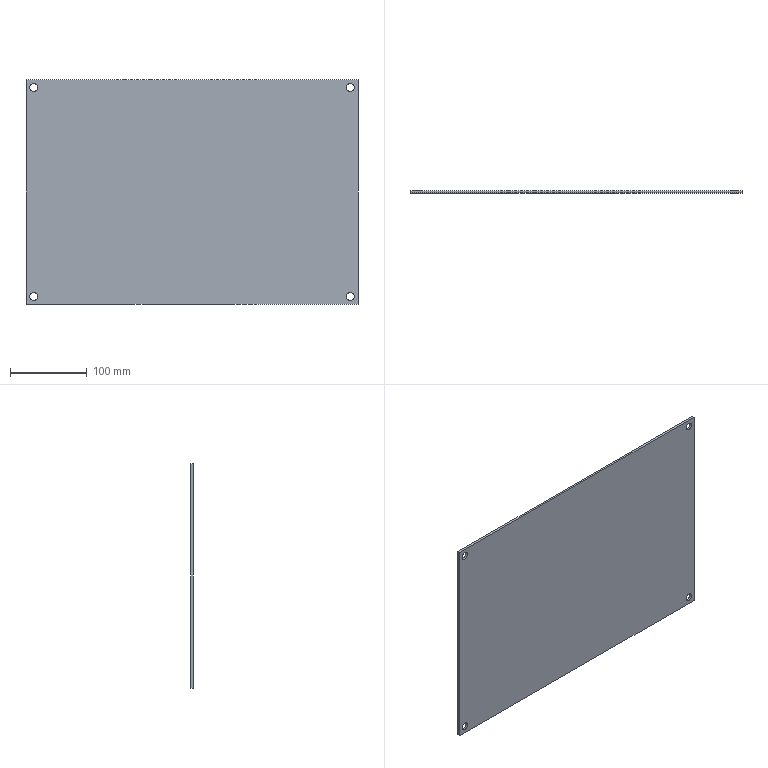Component | SolidWorks | FuelTank-1_FuelTankCap-1 | 1 solid | 14 faces | box 432 x 3 x 292 mm | volume 377490 mm3 | cylinder 8 | plane 6 | commonest cylinder face diameters 10 x8
build123d program:
from build123d import *

# Parameters (mm, degrees)
SKETCH1_W           = 432
SKETCH1_H           = 292
BOSS_EXTRUDE1_DEPTH = 3
SKETCH2_R           = 5
CUT_EXTRUDE1_DEPTH  = 3


with BuildPart() as part:
    # Sketch1 → Boss-Extrude1 (new body)
    with BuildSketch(Plane.XY):
        with Locations((151.422, -114.636)):
            Rectangle(SKETCH1_W, SKETCH1_H)
    extrude(amount=BOSS_EXTRUDE1_DEPTH)

    # Sketch2 → Cut-Extrude1 (cut)
    with BuildSketch(Plane.XY.offset(3)):
        with Locations((-54.578, 21.364)):
            Circle(SKETCH2_R)
        with Locations((357.422, 21.364)):
            Circle(SKETCH2_R)
        with Locations((357.422, -250.636)):
            Circle(SKETCH2_R)
        with Locations((-54.578, -250.636)):
            Circle(SKETCH2_R)
    extrude(amount=-CUT_EXTRUDE1_DEPTH, mode=Mode.SUBTRACT)


solid = part.part

# Placed as in the assembly
solid = solid.moved(Location((34.029, -468.434, -406.883), (90, 0, 0)))
STEP:
#1=CARTESIAN_POINT('',(-1.006,-18.442,-25.887));
#2=VERTEX_POINT('',#1);
#3=CARTESIAN_POINT('',(-0.6122,-18.442,-25.887));
#4=VERTEX_POINT('',#3);
#5=CARTESIAN_POINT('',(-0.809,-18.442,-25.887));
#6=DIRECTION('',(0.,-1.,-0.));
#7=DIRECTION('',(1.,0.,0.));
#8=AXIS2_PLACEMENT_3D('',#5,#6,#7);
#9=CIRCLE('',#8,0.1969);
#10=EDGE_CURVE('',#2,#4,#9,.T.);
#11=ORIENTED_EDGE('',*,*,#10,.F.);
#12=CARTESIAN_POINT('',(-1.006,-18.56,-25.887));
#13=VERTEX_POINT('',#12);
#14=CARTESIAN_POINT('',(-1.006,-18.442,-25.887));
#15=DIRECTION('',(0.,-1.,-0.));
#16=VECTOR('',#15,39.37);
#17=LINE('',#14,#16);
#18=EDGE_CURVE('',#2,#13,#17,.T.);
#19=ORIENTED_EDGE('',*,*,#18,.T.);
#20=CARTESIAN_POINT('',(-0.6122,-18.56,-25.887));
#21=VERTEX_POINT('',#20);
#22=CARTESIAN_POINT('',(-0.809,-18.56,-25.887));
#23=DIRECTION('',(0.,-1.,-0.));
#24=DIRECTION('',(1.,0.,0.));
#25=AXIS2_PLACEMENT_3D('',#22,#23,#24);
#26=CIRCLE('',#25,0.1969);
#27=EDGE_CURVE('',#13,#21,#26,.T.);
#28=ORIENTED_EDGE('',*,*,#27,.T.);
#29=CARTESIAN_POINT('',(-0.6122,-18.442,-25.887));
#30=DIRECTION('',(0.,-1.,-0.));
#31=VECTOR('',#30,39.37);
#32=LINE('',#29,#31);
#33=EDGE_CURVE('',#4,#21,#32,.T.);
#34=ORIENTED_EDGE('',*,*,#33,.F.);
#35=EDGE_LOOP('',(#11,#19,#28,#34));
#36=FACE_OUTER_BOUND('',#35,.T.);
#37=CARTESIAN_POINT('',(-0.809,-18.442,-25.887));
#38=DIRECTION('',(0.,-1.,-0.));
#39=DIRECTION('',(1.,0.,0.));
#40=AXIS2_PLACEMENT_3D('',#37,#38,#39);
#41=CYLINDRICAL_SURFACE('',#40,0.1969);
#42=ADVANCED_FACE('',(#36),#41,.F.);
#43=CARTESIAN_POINT('',(15.215,-18.442,-25.887));
#44=VERTEX_POINT('',#43);
#45=CARTESIAN_POINT('',(15.608,-18.442,-25.887));
#46=VERTEX_POINT('',#45);
#47=CARTESIAN_POINT('',(15.411,-18.442,-25.887));
#48=DIRECTION('',(0.,-1.,-0.));
#49=DIRECTION('',(1.,0.,0.));
#50=AXIS2_PLACEMENT_3D('',#47,#48,#49);
#51=CIRCLE('',#50,0.1969);
#52=EDGE_CURVE('',#44,#46,#51,.T.);
#53=ORIENTED_EDGE('',*,*,#52,.F.);
#54=CARTESIAN_POINT('',(15.215,-18.56,-25.887));
#55=VERTEX_POINT('',#54);
#56=CARTESIAN_POINT('',(15.215,-18.442,-25.887));
#57=DIRECTION('',(0.,-1.,-0.));
#58=VECTOR('',#57,39.37);
#59=LINE('',#56,#58);
#60=EDGE_CURVE('',#44,#55,#59,.T.);
#61=ORIENTED_EDGE('',*,*,#60,.T.);
#62=CARTESIAN_POINT('',(15.608,-18.56,-25.887));
#63=VERTEX_POINT('',#62);
#64=CARTESIAN_POINT('',(15.411,-18.56,-25.887));
#65=DIRECTION('',(0.,-1.,-0.));
#66=DIRECTION('',(1.,0.,0.));
#67=AXIS2_PLACEMENT_3D('',#64,#65,#66);
#68=CIRCLE('',#67,0.1969);
#69=EDGE_CURVE('',#55,#63,#68,.T.);
#70=ORIENTED_EDGE('',*,*,#69,.T.);
#71=CARTESIAN_POINT('',(15.608,-18.442,-25.887));
#72=DIRECTION('',(0.,-1.,-0.));
#73=VECTOR('',#72,39.37);
#74=LINE('',#71,#73);
#75=EDGE_CURVE('',#46,#63,#74,.T.);
#76=ORIENTED_EDGE('',*,*,#75,.F.);
#77=EDGE_LOOP('',(#53,#61,#70,#76));
#78=FACE_OUTER_BOUND('',#77,.T.);
#79=CARTESIAN_POINT('',(15.411,-18.442,-25.887));
#80=DIRECTION('',(0.,-1.,-0.));
#81=DIRECTION('',(1.,0.,0.));
#82=AXIS2_PLACEMENT_3D('',#79,#80,#81);
#83=CYLINDRICAL_SURFACE('',#82,0.1969);
#84=ADVANCED_FACE('',(#78),#83,.F.);
#85=CARTESIAN_POINT('',(15.215,-18.442,-15.178));
#86=VERTEX_POINT('',#85);
#87=CARTESIAN_POINT('',(15.608,-18.442,-15.178));
#88=VERTEX_POINT('',#87);
#89=CARTESIAN_POINT('',(15.411,-18.442,-15.178));
#90=DIRECTION('',(0.,-1.,-0.));
#91=DIRECTION('',(1.,0.,0.));
#92=AXIS2_PLACEMENT_3D('',#89,#90,#91);
#93=CIRCLE('',#92,0.1969);
#94=EDGE_CURVE('',#86,#88,#93,.T.);
#95=ORIENTED_EDGE('',*,*,#94,.F.);
#96=CARTESIAN_POINT('',(15.215,-18.56,-15.178));
#97=VERTEX_POINT('',#96);
#98=CARTESIAN_POINT('',(15.215,-18.442,-15.178));
#99=DIRECTION('',(0.,-1.,-0.));
#100=VECTOR('',#99,39.37);
#101=LINE('',#98,#100);
#102=EDGE_CURVE('',#86,#97,#101,.T.);
#103=ORIENTED_EDGE('',*,*,#102,.T.);
#104=CARTESIAN_POINT('',(15.608,-18.56,-15.178));
#105=VERTEX_POINT('',#104);
#106=CARTESIAN_POINT('',(15.411,-18.56,-15.178));
#107=DIRECTION('',(0.,-1.,-0.));
#108=DIRECTION('',(1.,0.,0.));
#109=AXIS2_PLACEMENT_3D('',#106,#107,#108);
#110=CIRCLE('',#109,0.1969);
#111=EDGE_CURVE('',#97,#105,#110,.T.);
#112=ORIENTED_EDGE('',*,*,#111,.T.);
#113=CARTESIAN_POINT('',(15.608,-18.442,-15.178));
#114=DIRECTION('',(0.,-1.,-0.));
#115=VECTOR('',#114,39.37);
#116=LINE('',#113,#115);
#117=EDGE_CURVE('',#88,#105,#116,.T.);
#118=ORIENTED_EDGE('',*,*,#117,.F.);
#119=EDGE_LOOP('',(#95,#103,#112,#118));
#120=FACE_OUTER_BOUND('',#119,.T.);
#121=CARTESIAN_POINT('',(15.411,-18.442,-15.178));
#122=DIRECTION('',(0.,-1.,-0.));
#123=DIRECTION('',(1.,0.,0.));
#124=AXIS2_PLACEMENT_3D('',#121,#122,#123);
#125=CYLINDRICAL_SURFACE('',#124,0.1969);
#126=ADVANCED_FACE('',(#120),#125,.F.);
#127=CARTESIAN_POINT('',(-1.006,-18.442,-15.178));
#128=VERTEX_POINT('',#127);
#129=CARTESIAN_POINT('',(-0.6122,-18.442,-15.178));
#130=VERTEX_POINT('',#129);
#131=CARTESIAN_POINT('',(-0.809,-18.442,-15.178));
#132=DIRECTION('',(0.,-1.,-0.));
#133=DIRECTION('',(1.,0.,0.));
#134=AXIS2_PLACEMENT_3D('',#131,#132,#133);
#135=CIRCLE('',#134,0.1969);
#136=EDGE_CURVE('',#128,#130,#135,.T.);
#137=ORIENTED_EDGE('',*,*,#136,.F.);
#138=CARTESIAN_POINT('',(-1.006,-18.56,-15.178));
#139=VERTEX_POINT('',#138);
#140=CARTESIAN_POINT('',(-1.006,-18.442,-15.178));
#141=DIRECTION('',(0.,-1.,-0.));
#142=VECTOR('',#141,39.37);
#143=LINE('',#140,#142);
#144=EDGE_CURVE('',#128,#139,#143,.T.);
#145=ORIENTED_EDGE('',*,*,#144,.T.);
#146=CARTESIAN_POINT('',(-0.6122,-18.56,-15.178));
#147=VERTEX_POINT('',#146);
#148=CARTESIAN_POINT('',(-0.809,-18.56,-15.178));
#149=DIRECTION('',(0.,-1.,-0.));
#150=DIRECTION('',(1.,0.,0.));
#151=AXIS2_PLACEMENT_3D('',#148,#149,#150);
#152=CIRCLE('',#151,0.1969);
#153=EDGE_CURVE('',#139,#147,#152,.T.);
#154=ORIENTED_EDGE('',*,*,#153,.T.);
#155=CARTESIAN_POINT('',(-0.6122,-18.442,-15.178));
#156=DIRECTION('',(0.,-1.,-0.));
#157=VECTOR('',#156,39.37);
#158=LINE('',#155,#157);
#159=EDGE_CURVE('',#130,#147,#158,.T.);
#160=ORIENTED_EDGE('',*,*,#159,.F.);
#161=EDGE_LOOP('',(#137,#145,#154,#160));
#162=FACE_OUTER_BOUND('',#161,.T.);
#163=CARTESIAN_POINT('',(-0.809,-18.442,-15.178));
#164=DIRECTION('',(0.,-1.,-0.));
#165=DIRECTION('',(1.,0.,0.));
#166=AXIS2_PLACEMENT_3D('',#163,#164,#165);
#167=CYLINDRICAL_SURFACE('',#166,0.1969);
#168=ADVANCED_FACE('',(#162),#167,.F.);
#169=CARTESIAN_POINT('',(-1.203,-18.442,-14.784));
#170=VERTEX_POINT('',#169);
#171=CARTESIAN_POINT('',(-1.203,-18.442,-26.28));
#172=VERTEX_POINT('',#171);
#173=CARTESIAN_POINT('',(-1.203,-18.442,-14.784));
#174=DIRECTION('',(0.,0.,-1.));
#175=VECTOR('',#174,39.37);
#176=LINE('',#173,#175);
#177=EDGE_CURVE('',#170,#172,#176,.T.);
#178=ORIENTED_EDGE('',*,*,#177,.T.);
#179=CARTESIAN_POINT('',(-1.203,-18.56,-26.28));
#180=VERTEX_POINT('',#179);
#181=CARTESIAN_POINT('',(-1.203,-18.56,-26.28));
#182=DIRECTION('',(-0.,1.,0.));
#183=VECTOR('',#182,39.37);
#184=LINE('',#181,#183);
#185=EDGE_CURVE('',#180,#172,#184,.T.);
#186=ORIENTED_EDGE('',*,*,#185,.F.);
#187=CARTESIAN_POINT('',(-1.203,-18.56,-14.784));
#188=VERTEX_POINT('',#187);
#189=CARTESIAN_POINT('',(-1.203,-18.56,-14.784));
#190=DIRECTION('',(0.,0.,-1.));
#191=VECTOR('',#190,39.37);
#192=LINE('',#189,#191);
#193=EDGE_CURVE('',#188,#180,#192,.T.);
#194=ORIENTED_EDGE('',*,*,#193,.F.);
#195=CARTESIAN_POINT('',(-1.203,-18.56,-14.784));
#196=DIRECTION('',(-0.,1.,0.));
#197=VECTOR('',#196,39.37);
#198=LINE('',#195,#197);
#199=EDGE_CURVE('',#188,#170,#198,.T.);
#200=ORIENTED_EDGE('',*,*,#199,.T.);
#201=EDGE_LOOP('',(#178,#186,#194,#200));
#202=FACE_OUTER_BOUND('',#201,.T.);
#203=CARTESIAN_POINT('',(-1.203,-18.56,-14.784));
#204=DIRECTION('',(1.,0.,0.));
#205=DIRECTION('',(-0.,-0.,1.));
#206=AXIS2_PLACEMENT_3D('',#203,#204,#205);
#207=PLANE('',#206);
#208=ADVANCED_FACE('',(#202),#207,.F.);
#209=CARTESIAN_POINT('',(15.805,-18.442,-26.28));
#210=VERTEX_POINT('',#209);
#211=CARTESIAN_POINT('',(-1.203,-18.442,-26.28));
#212=DIRECTION('',(1.,0.,0.));
#213=VECTOR('',#212,39.37);
#214=LINE('',#211,#213);
#215=EDGE_CURVE('',#172,#210,#214,.T.);
#216=ORIENTED_EDGE('',*,*,#215,.T.);
#217=CARTESIAN_POINT('',(15.805,-18.56,-26.28));
#218=VERTEX_POINT('',#217);
#219=CARTESIAN_POINT('',(15.805,-18.56,-26.28));
#220=DIRECTION('',(-0.,1.,0.));
#221=VECTOR('',#220,39.37);
#222=LINE('',#219,#221);
#223=EDGE_CURVE('',#218,#210,#222,.T.);
#224=ORIENTED_EDGE('',*,*,#223,.F.);
#225=CARTESIAN_POINT('',(-1.203,-18.56,-26.28));
#226=DIRECTION('',(1.,0.,0.));
#227=VECTOR('',#226,39.37);
#228=LINE('',#225,#227);
#229=EDGE_CURVE('',#180,#218,#228,.T.);
#230=ORIENTED_EDGE('',*,*,#229,.F.);
#231=ORIENTED_EDGE('',*,*,#185,.T.);
#232=EDGE_LOOP('',(#216,#224,#230,#231));
#233=FACE_OUTER_BOUND('',#232,.T.);
#234=CARTESIAN_POINT('',(-1.203,-18.56,-26.28));
#235=DIRECTION('',(-0.,-0.,1.));
#236=DIRECTION('',(0.,-1.,-0.));
#237=AXIS2_PLACEMENT_3D('',#234,#235,#236);
#238=PLANE('',#237);
#239=ADVANCED_FACE('',(#233),#238,.F.);
#240=CARTESIAN_POINT('',(15.805,-18.442,-14.784));
#241=VERTEX_POINT('',#240);
#242=CARTESIAN_POINT('',(15.805,-18.442,-14.784));
#243=DIRECTION('',(-0.,-0.,1.));
#244=VECTOR('',#243,39.37);
#245=LINE('',#242,#244);
#246=EDGE_CURVE('',#210,#241,#245,.T.);
#247=ORIENTED_EDGE('',*,*,#246,.T.);
#248=CARTESIAN_POINT('',(15.805,-18.56,-14.784));
#249=VERTEX_POINT('',#248);
#250=CARTESIAN_POINT('',(15.805,-18.56,-14.784));
#251=DIRECTION('',(-0.,1.,0.));
#252=VECTOR('',#251,39.37);
#253=LINE('',#250,#252);
#254=EDGE_CURVE('',#249,#241,#253,.T.);
#255=ORIENTED_EDGE('',*,*,#254,.F.);
#256=CARTESIAN_POINT('',(15.805,-18.56,-14.784));
#257=DIRECTION('',(-0.,-0.,1.));
#258=VECTOR('',#257,39.37);
#259=LINE('',#256,#258);
#260=EDGE_CURVE('',#218,#249,#259,.T.);
#261=ORIENTED_EDGE('',*,*,#260,.F.);
#262=ORIENTED_EDGE('',*,*,#223,.T.);
#263=EDGE_LOOP('',(#247,#255,#261,#262));
#264=FACE_OUTER_BOUND('',#263,.T.);
#265=CARTESIAN_POINT('',(15.805,-18.56,-14.784));
#266=DIRECTION('',(-1.,-0.,-0.));
#267=DIRECTION('',(0.,0.,-1.));
#268=AXIS2_PLACEMENT_3D('',#265,#266,#267);
#269=PLANE('',#268);
#270=ADVANCED_FACE('',(#264),#269,.F.);
#271=CARTESIAN_POINT('',(-1.203,-18.442,-14.784));
#272=DIRECTION('',(-1.,-0.,-0.));
#273=VECTOR('',#272,39.37);
#274=LINE('',#271,#273);
#275=EDGE_CURVE('',#241,#170,#274,.T.);
#276=ORIENTED_EDGE('',*,*,#275,.T.);
#277=ORIENTED_EDGE('',*,*,#199,.F.);
#278=CARTESIAN_POINT('',(-1.203,-18.56,-14.784));
#279=DIRECTION('',(-1.,-0.,-0.));
#280=VECTOR('',#279,39.37);
#281=LINE('',#278,#280);
#282=EDGE_CURVE('',#249,#188,#281,.T.);
#283=ORIENTED_EDGE('',*,*,#282,.F.);
#284=ORIENTED_EDGE('',*,*,#254,.T.);
#285=EDGE_LOOP('',(#276,#277,#283,#284));
#286=FACE_OUTER_BOUND('',#285,.T.);
#287=CARTESIAN_POINT('',(-1.203,-18.56,-14.784));
#288=DIRECTION('',(0.,0.,-1.));
#289=DIRECTION('',(-0.,1.,0.));
#290=AXIS2_PLACEMENT_3D('',#287,#288,#289);
#291=PLANE('',#290);
#292=ADVANCED_FACE('',(#286),#291,.F.);
#293=CARTESIAN_POINT('',(-0.809,-18.56,-25.887));
#294=DIRECTION('',(0.,-1.,-0.));
#295=DIRECTION('',(1.,0.,0.));
#296=AXIS2_PLACEMENT_3D('',#293,#294,#295);
#297=CIRCLE('',#296,0.1969);
#298=EDGE_CURVE('',#21,#13,#297,.T.);
#299=ORIENTED_EDGE('',*,*,#298,.F.);
#300=ORIENTED_EDGE('',*,*,#27,.F.);
#301=EDGE_LOOP('',(#299,#300));
#302=FACE_BOUND('',#301,.T.);
#303=CARTESIAN_POINT('',(15.411,-18.56,-25.887));
#304=DIRECTION('',(0.,-1.,-0.));
#305=DIRECTION('',(1.,0.,0.));
#306=AXIS2_PLACEMENT_3D('',#303,#304,#305);
#307=CIRCLE('',#306,0.1969);
#308=EDGE_CURVE('',#63,#55,#307,.T.);
#309=ORIENTED_EDGE('',*,*,#308,.F.);
#310=ORIENTED_EDGE('',*,*,#69,.F.);
#311=EDGE_LOOP('',(#309,#310));
#312=FACE_BOUND('',#311,.T.);
#313=CARTESIAN_POINT('',(15.411,-18.56,-15.178));
#314=DIRECTION('',(0.,-1.,-0.));
#315=DIRECTION('',(1.,0.,0.));
#316=AXIS2_PLACEMENT_3D('',#313,#314,#315);
#317=CIRCLE('',#316,0.1969);
#318=EDGE_CURVE('',#105,#97,#317,.T.);
#319=ORIENTED_EDGE('',*,*,#318,.F.);
#320=ORIENTED_EDGE('',*,*,#111,.F.);
#321=EDGE_LOOP('',(#319,#320));
#322=FACE_BOUND('',#321,.T.);
#323=CARTESIAN_POINT('',(-0.809,-18.56,-15.178));
#324=DIRECTION('',(0.,-1.,-0.));
#325=DIRECTION('',(1.,0.,0.));
#326=AXIS2_PLACEMENT_3D('',#323,#324,#325);
#327=CIRCLE('',#326,0.1969);
#328=EDGE_CURVE('',#147,#139,#327,.T.);
#329=ORIENTED_EDGE('',*,*,#328,.F.);
#330=ORIENTED_EDGE('',*,*,#153,.F.);
#331=EDGE_LOOP('',(#329,#330));
#332=FACE_BOUND('',#331,.T.);
#333=ORIENTED_EDGE('',*,*,#193,.T.);
#334=ORIENTED_EDGE('',*,*,#229,.T.);
#335=ORIENTED_EDGE('',*,*,#260,.T.);
#336=ORIENTED_EDGE('',*,*,#282,.T.);
#337=EDGE_LOOP('',(#333,#334,#335,#336));
#338=FACE_OUTER_BOUND('',#337,.T.);
#339=CARTESIAN_POINT('',(1.34,-18.56,-16.019));
#340=DIRECTION('',(0.,-1.,-0.));
#341=DIRECTION('',(1.,0.,0.));
#342=AXIS2_PLACEMENT_3D('',#339,#340,#341);
#343=PLANE('',#342);
#344=ADVANCED_FACE('',(#302,#312,#322,#332,#338),#343,.T.);
#345=CARTESIAN_POINT('',(-0.809,-18.442,-25.887));
#346=DIRECTION('',(0.,-1.,-0.));
#347=DIRECTION('',(1.,0.,0.));
#348=AXIS2_PLACEMENT_3D('',#345,#346,#347);
#349=CIRCLE('',#348,0.1969);
#350=EDGE_CURVE('',#4,#2,#349,.T.);
#351=ORIENTED_EDGE('',*,*,#350,.T.);
#352=ORIENTED_EDGE('',*,*,#10,.T.);
#353=EDGE_LOOP('',(#351,#352));
#354=FACE_BOUND('',#353,.T.);
#355=CARTESIAN_POINT('',(15.411,-18.442,-25.887));
#356=DIRECTION('',(0.,-1.,-0.));
#357=DIRECTION('',(1.,0.,0.));
#358=AXIS2_PLACEMENT_3D('',#355,#356,#357);
#359=CIRCLE('',#358,0.1969);
#360=EDGE_CURVE('',#46,#44,#359,.T.);
#361=ORIENTED_EDGE('',*,*,#360,.T.);
#362=ORIENTED_EDGE('',*,*,#52,.T.);
#363=EDGE_LOOP('',(#361,#362));
#364=FACE_BOUND('',#363,.T.);
#365=CARTESIAN_POINT('',(15.411,-18.442,-15.178));
#366=DIRECTION('',(0.,-1.,-0.));
#367=DIRECTION('',(1.,0.,0.));
#368=AXIS2_PLACEMENT_3D('',#365,#366,#367);
#369=CIRCLE('',#368,0.1969);
#370=EDGE_CURVE('',#88,#86,#369,.T.);
#371=ORIENTED_EDGE('',*,*,#370,.T.);
#372=ORIENTED_EDGE('',*,*,#94,.T.);
#373=EDGE_LOOP('',(#371,#372));
#374=FACE_BOUND('',#373,.T.);
#375=CARTESIAN_POINT('',(-0.809,-18.442,-15.178));
#376=DIRECTION('',(0.,-1.,-0.));
#377=DIRECTION('',(1.,0.,0.));
#378=AXIS2_PLACEMENT_3D('',#375,#376,#377);
#379=CIRCLE('',#378,0.1969);
#380=EDGE_CURVE('',#130,#128,#379,.T.);
#381=ORIENTED_EDGE('',*,*,#380,.T.);
#382=ORIENTED_EDGE('',*,*,#136,.T.);
#383=EDGE_LOOP('',(#381,#382));
#384=FACE_BOUND('',#383,.T.);
#385=ORIENTED_EDGE('',*,*,#177,.F.);
#386=ORIENTED_EDGE('',*,*,#275,.F.);
#387=ORIENTED_EDGE('',*,*,#246,.F.);
#388=ORIENTED_EDGE('',*,*,#215,.F.);
#389=EDGE_LOOP('',(#385,#386,#387,#388));
#390=FACE_OUTER_BOUND('',#389,.T.);
#391=CARTESIAN_POINT('',(1.34,-18.442,-16.019));
#392=DIRECTION('',(0.,-1.,-0.));
#393=DIRECTION('',(1.,0.,0.));
#394=AXIS2_PLACEMENT_3D('',#391,#392,#393);
#395=PLANE('',#394);
#396=ADVANCED_FACE('',(#354,#364,#374,#384,#390),#395,.F.);
#397=ORIENTED_EDGE('',*,*,#144,.F.);
#398=ORIENTED_EDGE('',*,*,#380,.F.);
#399=ORIENTED_EDGE('',*,*,#159,.T.);
#400=ORIENTED_EDGE('',*,*,#328,.T.);
#401=EDGE_LOOP('',(#397,#398,#399,#400));
#402=FACE_OUTER_BOUND('',#401,.T.);
#403=CARTESIAN_POINT('',(-0.809,-18.442,-15.178));
#404=DIRECTION('',(0.,-1.,-0.));
#405=DIRECTION('',(1.,0.,0.));
#406=AXIS2_PLACEMENT_3D('',#403,#404,#405);
#407=CYLINDRICAL_SURFACE('',#406,0.1969);
#408=ADVANCED_FACE('',(#402),#407,.F.);
#409=ORIENTED_EDGE('',*,*,#102,.F.);
#410=ORIENTED_EDGE('',*,*,#370,.F.);
#411=ORIENTED_EDGE('',*,*,#117,.T.);
#412=ORIENTED_EDGE('',*,*,#318,.T.);
#413=EDGE_LOOP('',(#409,#410,#411,#412));
#414=FACE_OUTER_BOUND('',#413,.T.);
#415=CARTESIAN_POINT('',(15.411,-18.442,-15.178));
#416=DIRECTION('',(0.,-1.,-0.));
#417=DIRECTION('',(1.,0.,0.));
#418=AXIS2_PLACEMENT_3D('',#415,#416,#417);
#419=CYLINDRICAL_SURFACE('',#418,0.1969);
#420=ADVANCED_FACE('',(#414),#419,.F.);
#421=ORIENTED_EDGE('',*,*,#60,.F.);
#422=ORIENTED_EDGE('',*,*,#360,.F.);
#423=ORIENTED_EDGE('',*,*,#75,.T.);
#424=ORIENTED_EDGE('',*,*,#308,.T.);
#425=EDGE_LOOP('',(#421,#422,#423,#424));
#426=FACE_OUTER_BOUND('',#425,.T.);
#427=CARTESIAN_POINT('',(15.411,-18.442,-25.887));
#428=DIRECTION('',(0.,-1.,-0.));
#429=DIRECTION('',(1.,0.,0.));
#430=AXIS2_PLACEMENT_3D('',#427,#428,#429);
#431=CYLINDRICAL_SURFACE('',#430,0.1969);
#432=ADVANCED_FACE('',(#426),#431,.F.);
#433=ORIENTED_EDGE('',*,*,#18,.F.);
#434=ORIENTED_EDGE('',*,*,#350,.F.);
#435=ORIENTED_EDGE('',*,*,#33,.T.);
#436=ORIENTED_EDGE('',*,*,#298,.T.);
#437=EDGE_LOOP('',(#433,#434,#435,#436));
#438=FACE_OUTER_BOUND('',#437,.T.);
#439=CARTESIAN_POINT('',(-0.809,-18.442,-25.887));
#440=DIRECTION('',(0.,-1.,-0.));
#441=DIRECTION('',(1.,0.,0.));
#442=AXIS2_PLACEMENT_3D('',#439,#440,#441);
#443=CYLINDRICAL_SURFACE('',#442,0.1969);
#444=ADVANCED_FACE('',(#438),#443,.F.);
#445=CLOSED_SHELL('',(#42,#84,#126,#168,#208,#239,#270,#292,#344,#396,#408,#420,#432,#444));
#446=MANIFOLD_SOLID_BREP('',#445);
#447=CARTESIAN_POINT('',(0.,0.,0.));
#448=DIRECTION('',(0.,0.,1.));
#449=DIRECTION('',(1.,0.,0.));
#450=AXIS2_PLACEMENT_3D('',#447,#448,#449);
#451=(LENGTH_UNIT()NAMED_UNIT(*)SI_UNIT($,.METRE.));
#452=LENGTH_MEASURE_WITH_UNIT(LENGTH_MEASURE(0.0254),#451);
#453=DIMENSIONAL_EXPONENTS(1.,0.,0.,0.,0.,0.,0.);
#454=(CONVERSION_BASED_UNIT('',#452)LENGTH_UNIT()NAMED_UNIT(#453));
#455=UNCERTAINTY_MEASURE_WITH_UNIT(LENGTH_MEASURE(0.00001),#454,'','');
#456=(NAMED_UNIT(*)PLANE_ANGLE_UNIT()SI_UNIT($,.RADIAN.));
#457=(NAMED_UNIT(*)SI_UNIT($,.STERADIAN.)SOLID_ANGLE_UNIT());
#458=(GEOMETRIC_REPRESENTATION_CONTEXT(3)GLOBAL_UNCERTAINTY_ASSIGNED_CONTEXT((#455))GLOBAL_UNIT_ASSIGNED_CONTEXT((#454,#456,#457))REPRESENTATION_CONTEXT('',''));
#459=ADVANCED_BREP_SHAPE_REPRESENTATION('',(#446,#450),#458);
#460=COLOUR_RGB('',0.7922,0.8196,0.9333);
#461=FILL_AREA_STYLE_COLOUR('',#460);
#462=FILL_AREA_STYLE('',(#461));
#463=SURFACE_STYLE_FILL_AREA(#462);
#464=SURFACE_SIDE_STYLE('',(#463));
#465=SURFACE_STYLE_USAGE(.BOTH.,#464);
#466=PRESENTATION_STYLE_ASSIGNMENT((#465));
#467=STYLED_ITEM('',(#466),#446);
#468=PRESENTATION_LAYER_ASSIGNMENT('','',(#467));
#469=(LENGTH_UNIT()NAMED_UNIT(*)SI_UNIT($,.METRE.));
#470=LENGTH_MEASURE_WITH_UNIT(LENGTH_MEASURE(0.0254),#469);
#471=DIMENSIONAL_EXPONENTS(1.,0.,0.,0.,0.,0.,0.);
#472=(CONVERSION_BASED_UNIT('',#470)LENGTH_UNIT()NAMED_UNIT(#471));
#473=UNCERTAINTY_MEASURE_WITH_UNIT(LENGTH_MEASURE(0.00001),#472,'','');
#474=(NAMED_UNIT(*)PLANE_ANGLE_UNIT()SI_UNIT($,.RADIAN.));
#475=(NAMED_UNIT(*)SI_UNIT($,.STERADIAN.)SOLID_ANGLE_UNIT());
#476=(GEOMETRIC_REPRESENTATION_CONTEXT(3)GLOBAL_UNCERTAINTY_ASSIGNED_CONTEXT((#473))GLOBAL_UNIT_ASSIGNED_CONTEXT((#472,#474,#475))REPRESENTATION_CONTEXT('',''));
#477=MECHANICAL_DESIGN_GEOMETRIC_PRESENTATION_REPRESENTATION('',(#467),#476);